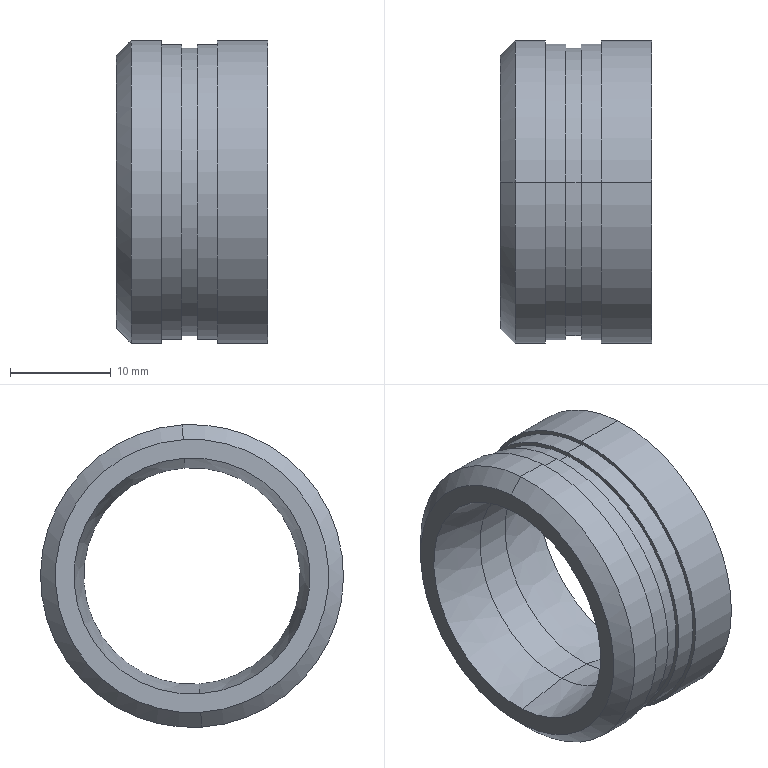Component | SolidWorks | 216InnerTubeAssembly-1_DampingSleeve-1 | 1 solid | 26 faces | box 15 x 30 x 30 mm | volume 4390 mm3 | cylinder 12 | cone 10 | plane 4 | commonest cylinder face diameters 30 x4 29.265 x2 28.514 x2 29.257 x2 21.449 x2 | material Polyurethane(11671)
build123d program:
from build123d import *


with BuildPart() as part:
    # Model → Revolve1 (revolve)
    with BuildSketch(Plane.XY, mode=Mode.PRIVATE) as revolve1_sk:
        Polygon((1.544, 15.169), (0.07655, 13.701), (0.07655, 11.863), (5.577, 10.893), (9.077, 10.893), (15.077, 12.169), (15.077, 15.169), (10.077, 15.169), (10.077, 14.797), (8.077, 14.797), (8.077, 14.426), (6.577, 14.426), (6.578, 14.801), (4.544, 14.801), (4.544, 15.169), align=None)
    revolve(revolve1_sk.sketch.rotate(Axis((0.08037, 0.1686, 0), (1, 0, 0)), 90), axis=Axis((0.08037, 0.1686, 0), (1, 0, 0)))


solid = part.part

# Placed as in the assembly
solid = solid.moved(Location((658.502, -0.1686, 0), (0, 0, 0)))
STEP:
#1=COLOUR_RGB('',0.7922,0.8196,0.9333);
#2=FILL_AREA_STYLE_COLOUR('',#1);
#3=FILL_AREA_STYLE('',(#2));
#4=SURFACE_STYLE_FILL_AREA(#3);
#5=SURFACE_SIDE_STYLE('',(#4));
#6=SURFACE_STYLE_USAGE(.BOTH.,#5);
#7=PRESENTATION_STYLE_ASSIGNMENT((#6));
#8=CARTESIAN_POINT('',(26.104,0.03778,0.5893));
#9=VERTEX_POINT('',#8);
#10=CARTESIAN_POINT('',(26.104,-0.03778,-0.5893));
#11=VERTEX_POINT('',#10);
#12=CARTESIAN_POINT('',(26.104,-0.,0.));
#13=DIRECTION('',(-1.,-0.,0.));
#14=DIRECTION('',(0.,0.06397,0.998));
#15=AXIS2_PLACEMENT_3D('',#12,#13,#14);
#16=CIRCLE('',#15,0.5906);
#17=EDGE_CURVE('',#9,#11,#16,.T.);
#18=ORIENTED_EDGE('',*,*,#17,.T.);
#19=CARTESIAN_POINT('',(25.986,-0.03778,-0.5893));
#20=VERTEX_POINT('',#19);
#21=CARTESIAN_POINT('',(25.928,-0.03778,-0.5893));
#22=DIRECTION('',(-1.,-0.,0.));
#23=VECTOR('',#22,39.37);
#24=LINE('',#21,#23);
#25=EDGE_CURVE('',#11,#20,#24,.T.);
#26=ORIENTED_EDGE('',*,*,#25,.T.);
#27=CARTESIAN_POINT('',(25.986,0.03778,0.5893));
#28=VERTEX_POINT('',#27);
#29=CARTESIAN_POINT('',(25.986,-0.,0.));
#30=DIRECTION('',(-1.,-0.,0.));
#31=DIRECTION('',(0.,0.06397,0.998));
#32=AXIS2_PLACEMENT_3D('',#29,#30,#31);
#33=CIRCLE('',#32,0.5906);
#34=EDGE_CURVE('',#28,#20,#33,.T.);
#35=ORIENTED_EDGE('',*,*,#34,.F.);
#36=CARTESIAN_POINT('',(25.928,0.03778,0.5893));
#37=DIRECTION('',(-1.,-0.,0.));
#38=VECTOR('',#37,39.37);
#39=LINE('',#36,#38);
#40=EDGE_CURVE('',#9,#28,#39,.T.);
#41=ORIENTED_EDGE('',*,*,#40,.F.);
#42=EDGE_LOOP('',(#18,#26,#35,#41));
#43=FACE_OUTER_BOUND('',#42,.T.);
#44=CARTESIAN_POINT('',(25.928,-0.,0.));
#45=DIRECTION('',(-1.,-0.,0.));
#46=DIRECTION('',(0.,0.06397,0.998));
#47=AXIS2_PLACEMENT_3D('',#44,#45,#46);
#48=CYLINDRICAL_SURFACE('',#47,0.5906);
#49=ADVANCED_FACE('',(#43),#48,.T.);
#50=CARTESIAN_POINT('',(26.184,0.03685,0.5749));
#51=VERTEX_POINT('',#50);
#52=CARTESIAN_POINT('',(26.184,-0.03685,-0.5749));
#53=VERTEX_POINT('',#52);
#54=CARTESIAN_POINT('',(26.184,-0.,0.));
#55=DIRECTION('',(-1.,-0.,0.));
#56=DIRECTION('',(0.,0.06397,0.998));
#57=AXIS2_PLACEMENT_3D('',#54,#55,#56);
#58=CIRCLE('',#57,0.5761);
#59=EDGE_CURVE('',#51,#53,#58,.T.);
#60=ORIENTED_EDGE('',*,*,#59,.T.);
#61=CARTESIAN_POINT('',(26.104,-0.03685,-0.5749));
#62=VERTEX_POINT('',#61);
#63=CARTESIAN_POINT('',(25.928,-0.03685,-0.5749));
#64=DIRECTION('',(-1.,-0.,0.));
#65=VECTOR('',#64,39.37);
#66=LINE('',#63,#65);
#67=EDGE_CURVE('',#53,#62,#66,.T.);
#68=ORIENTED_EDGE('',*,*,#67,.T.);
#69=CARTESIAN_POINT('',(26.104,0.03685,0.5749));
#70=VERTEX_POINT('',#69);
#71=CARTESIAN_POINT('',(26.104,-0.,0.));
#72=DIRECTION('',(-1.,-0.,0.));
#73=DIRECTION('',(0.,0.06397,0.998));
#74=AXIS2_PLACEMENT_3D('',#71,#72,#73);
#75=CIRCLE('',#74,0.5761);
#76=EDGE_CURVE('',#70,#62,#75,.T.);
#77=ORIENTED_EDGE('',*,*,#76,.F.);
#78=CARTESIAN_POINT('',(25.928,0.03685,0.5749));
#79=DIRECTION('',(-1.,-0.,0.));
#80=VECTOR('',#79,39.37);
#81=LINE('',#78,#80);
#82=EDGE_CURVE('',#51,#70,#81,.T.);
#83=ORIENTED_EDGE('',*,*,#82,.F.);
#84=EDGE_LOOP('',(#60,#68,#77,#83));
#85=FACE_OUTER_BOUND('',#84,.T.);
#86=CARTESIAN_POINT('',(25.928,-0.,0.));
#87=DIRECTION('',(-1.,-0.,0.));
#88=DIRECTION('',(0.,0.06397,0.998));
#89=AXIS2_PLACEMENT_3D('',#86,#87,#88);
#90=CYLINDRICAL_SURFACE('',#89,0.5761);
#91=ADVANCED_FACE('',(#85),#90,.T.);
#92=CARTESIAN_POINT('',(26.184,-0.03591,-0.5602));
#93=VERTEX_POINT('',#92);
#94=CARTESIAN_POINT('',(26.184,0.03591,0.5602));
#95=VERTEX_POINT('',#94);
#96=CARTESIAN_POINT('',(26.184,-0.,0.));
#97=DIRECTION('',(-1.,-0.,0.));
#98=DIRECTION('',(0.,0.06397,0.998));
#99=AXIS2_PLACEMENT_3D('',#96,#97,#98);
#100=CIRCLE('',#99,0.5613);
#101=EDGE_CURVE('',#93,#95,#100,.T.);
#102=ORIENTED_EDGE('',*,*,#101,.T.);
#103=CARTESIAN_POINT('',(26.184,0.03591,0.5602));
#104=DIRECTION('',(0.001262,0.06397,0.998));
#105=VECTOR('',#104,39.37);
#106=LINE('',#103,#105);
#107=EDGE_CURVE('',#95,#51,#106,.T.);
#108=ORIENTED_EDGE('',*,*,#107,.T.);
#109=CARTESIAN_POINT('',(26.184,-0.,0.));
#110=DIRECTION('',(-1.,-0.,0.));
#111=DIRECTION('',(0.,0.06397,0.998));
#112=AXIS2_PLACEMENT_3D('',#109,#110,#111);
#113=CIRCLE('',#112,0.5761);
#114=EDGE_CURVE('',#53,#51,#113,.T.);
#115=ORIENTED_EDGE('',*,*,#114,.F.);
#116=CARTESIAN_POINT('',(26.184,-0.03591,-0.5602));
#117=DIRECTION('',(0.001262,-0.06397,-0.998));
#118=VECTOR('',#117,39.37);
#119=LINE('',#116,#118);
#120=EDGE_CURVE('',#93,#53,#119,.T.);
#121=ORIENTED_EDGE('',*,*,#120,.F.);
#122=EDGE_LOOP('',(#102,#108,#115,#121));
#123=FACE_OUTER_BOUND('',#122,.T.);
#124=CARTESIAN_POINT('',(26.184,-0.,0.));
#125=DIRECTION('',(1.,0.,-0.));
#126=DIRECTION('',(0.,-0.06397,-0.998));
#127=AXIS2_PLACEMENT_3D('',#124,#125,#126);
#128=CONICAL_SURFACE('',#127,0.5613,1.57);
#129=ADVANCED_FACE('',(#123),#128,.F.);
#130=CARTESIAN_POINT('',(26.243,0.03591,0.5602));
#131=VERTEX_POINT('',#130);
#132=CARTESIAN_POINT('',(26.243,-0.03591,-0.5602));
#133=VERTEX_POINT('',#132);
#134=CARTESIAN_POINT('',(26.243,-0.,0.));
#135=DIRECTION('',(-1.,-0.,0.));
#136=DIRECTION('',(0.,0.06397,0.998));
#137=AXIS2_PLACEMENT_3D('',#134,#135,#136);
#138=CIRCLE('',#137,0.5613);
#139=EDGE_CURVE('',#131,#133,#138,.T.);
#140=ORIENTED_EDGE('',*,*,#139,.T.);
#141=CARTESIAN_POINT('',(25.928,-0.03591,-0.5602));
#142=DIRECTION('',(-1.,-0.,0.));
#143=VECTOR('',#142,39.37);
#144=LINE('',#141,#143);
#145=EDGE_CURVE('',#133,#93,#144,.T.);
#146=ORIENTED_EDGE('',*,*,#145,.T.);
#147=CARTESIAN_POINT('',(26.184,-0.,0.));
#148=DIRECTION('',(-1.,-0.,0.));
#149=DIRECTION('',(0.,0.06397,0.998));
#150=AXIS2_PLACEMENT_3D('',#147,#148,#149);
#151=CIRCLE('',#150,0.5613);
#152=EDGE_CURVE('',#95,#93,#151,.T.);
#153=ORIENTED_EDGE('',*,*,#152,.F.);
#154=CARTESIAN_POINT('',(25.928,0.03591,0.5602));
#155=DIRECTION('',(-1.,-0.,0.));
#156=VECTOR('',#155,39.37);
#157=LINE('',#154,#156);
#158=EDGE_CURVE('',#131,#95,#157,.T.);
#159=ORIENTED_EDGE('',*,*,#158,.F.);
#160=EDGE_LOOP('',(#140,#146,#153,#159));
#161=FACE_OUTER_BOUND('',#160,.T.);
#162=CARTESIAN_POINT('',(25.928,-0.,0.));
#163=DIRECTION('',(-1.,-0.,0.));
#164=DIRECTION('',(0.,0.06397,0.998));
#165=AXIS2_PLACEMENT_3D('',#162,#163,#164);
#166=CYLINDRICAL_SURFACE('',#165,0.5613);
#167=ADVANCED_FACE('',(#161),#166,.T.);
#168=CARTESIAN_POINT('',(26.322,0.03684,0.5747));
#169=VERTEX_POINT('',#168);
#170=CARTESIAN_POINT('',(26.322,-0.03684,-0.5747));
#171=VERTEX_POINT('',#170);
#172=CARTESIAN_POINT('',(26.322,-0.,0.));
#173=DIRECTION('',(-1.,-0.,0.));
#174=DIRECTION('',(0.,0.06397,0.998));
#175=AXIS2_PLACEMENT_3D('',#172,#173,#174);
#176=CIRCLE('',#175,0.5759);
#177=EDGE_CURVE('',#169,#171,#176,.T.);
#178=ORIENTED_EDGE('',*,*,#177,.T.);
#179=CARTESIAN_POINT('',(26.243,-0.03684,-0.5747));
#180=VERTEX_POINT('',#179);
#181=CARTESIAN_POINT('',(25.928,-0.03684,-0.5747));
#182=DIRECTION('',(-1.,-0.,0.));
#183=VECTOR('',#182,39.37);
#184=LINE('',#181,#183);
#185=EDGE_CURVE('',#171,#180,#184,.T.);
#186=ORIENTED_EDGE('',*,*,#185,.T.);
#187=CARTESIAN_POINT('',(26.243,0.03684,0.5747));
#188=VERTEX_POINT('',#187);
#189=CARTESIAN_POINT('',(26.243,-0.,0.));
#190=DIRECTION('',(-1.,-0.,0.));
#191=DIRECTION('',(0.,0.06397,0.998));
#192=AXIS2_PLACEMENT_3D('',#189,#190,#191);
#193=CIRCLE('',#192,0.5759);
#194=EDGE_CURVE('',#188,#180,#193,.T.);
#195=ORIENTED_EDGE('',*,*,#194,.F.);
#196=CARTESIAN_POINT('',(25.928,0.03684,0.5747));
#197=DIRECTION('',(-1.,-0.,0.));
#198=VECTOR('',#197,39.37);
#199=LINE('',#196,#198);
#200=EDGE_CURVE('',#169,#188,#199,.T.);
#201=ORIENTED_EDGE('',*,*,#200,.F.);
#202=EDGE_LOOP('',(#178,#186,#195,#201));
#203=FACE_OUTER_BOUND('',#202,.T.);
#204=CARTESIAN_POINT('',(25.928,-0.,0.));
#205=DIRECTION('',(-1.,-0.,0.));
#206=DIRECTION('',(0.,0.06397,0.998));
#207=AXIS2_PLACEMENT_3D('',#204,#205,#206);
#208=CYLINDRICAL_SURFACE('',#207,0.5759);
#209=ADVANCED_FACE('',(#203),#208,.T.);
#210=CARTESIAN_POINT('',(26.322,-0.,0.));
#211=DIRECTION('',(-1.,-0.,0.));
#212=DIRECTION('',(0.,0.06397,0.998));
#213=AXIS2_PLACEMENT_3D('',#210,#211,#212);
#214=CIRCLE('',#213,0.5759);
#215=EDGE_CURVE('',#171,#169,#214,.T.);
#216=ORIENTED_EDGE('',*,*,#215,.F.);
#217=CARTESIAN_POINT('',(26.322,-0.03778,-0.5893));
#218=VERTEX_POINT('',#217);
#219=CARTESIAN_POINT('',(26.322,-0.03684,-0.5747));
#220=DIRECTION('',(-0.002523,-0.06397,-0.9979));
#221=VECTOR('',#220,39.37);
#222=LINE('',#219,#221);
#223=EDGE_CURVE('',#171,#218,#222,.T.);
#224=ORIENTED_EDGE('',*,*,#223,.T.);
#225=CARTESIAN_POINT('',(26.322,0.03778,0.5893));
#226=VERTEX_POINT('',#225);
#227=CARTESIAN_POINT('',(26.322,-0.,0.));
#228=DIRECTION('',(-1.,-0.,0.));
#229=DIRECTION('',(0.,0.06397,0.998));
#230=AXIS2_PLACEMENT_3D('',#227,#228,#229);
#231=CIRCLE('',#230,0.5906);
#232=EDGE_CURVE('',#218,#226,#231,.T.);
#233=ORIENTED_EDGE('',*,*,#232,.T.);
#234=CARTESIAN_POINT('',(26.322,0.03684,0.5747));
#235=DIRECTION('',(-0.002523,0.06397,0.9979));
#236=VECTOR('',#235,39.37);
#237=LINE('',#234,#236);
#238=EDGE_CURVE('',#169,#226,#237,.T.);
#239=ORIENTED_EDGE('',*,*,#238,.F.);
#240=EDGE_LOOP('',(#216,#224,#233,#239));
#241=FACE_OUTER_BOUND('',#240,.T.);
#242=CARTESIAN_POINT('',(26.322,-0.,0.));
#243=DIRECTION('',(-1.,-0.,0.));
#244=DIRECTION('',(0.,0.06397,0.998));
#245=AXIS2_PLACEMENT_3D('',#242,#243,#244);
#246=CONICAL_SURFACE('',#245,0.5759,1.568);
#247=ADVANCED_FACE('',(#241),#246,.F.);
#248=CARTESIAN_POINT('',(26.519,0.03778,0.5893));
#249=VERTEX_POINT('',#248);
#250=CARTESIAN_POINT('',(26.519,-0.03778,-0.5893));
#251=VERTEX_POINT('',#250);
#252=CARTESIAN_POINT('',(26.519,-0.,0.));
#253=DIRECTION('',(-1.,-0.,0.));
#254=DIRECTION('',(0.,0.06397,0.998));
#255=AXIS2_PLACEMENT_3D('',#252,#253,#254);
#256=CIRCLE('',#255,0.5906);
#257=EDGE_CURVE('',#249,#251,#256,.T.);
#258=ORIENTED_EDGE('',*,*,#257,.T.);
#259=CARTESIAN_POINT('',(25.928,-0.03778,-0.5893));
#260=DIRECTION('',(-1.,-0.,0.));
#261=VECTOR('',#260,39.37);
#262=LINE('',#259,#261);
#263=EDGE_CURVE('',#251,#218,#262,.T.);
#264=ORIENTED_EDGE('',*,*,#263,.T.);
#265=CARTESIAN_POINT('',(26.322,-0.,0.));
#266=DIRECTION('',(-1.,-0.,0.));
#267=DIRECTION('',(0.,0.06397,0.998));
#268=AXIS2_PLACEMENT_3D('',#265,#266,#267);
#269=CIRCLE('',#268,0.5906);
#270=EDGE_CURVE('',#226,#218,#269,.T.);
#271=ORIENTED_EDGE('',*,*,#270,.F.);
#272=CARTESIAN_POINT('',(25.928,0.03778,0.5893));
#273=DIRECTION('',(-1.,-0.,0.));
#274=VECTOR('',#273,39.37);
#275=LINE('',#272,#274);
#276=EDGE_CURVE('',#249,#226,#275,.T.);
#277=ORIENTED_EDGE('',*,*,#276,.F.);
#278=EDGE_LOOP('',(#258,#264,#271,#277));
#279=FACE_OUTER_BOUND('',#278,.T.);
#280=CARTESIAN_POINT('',(25.928,-0.,0.));
#281=DIRECTION('',(-1.,-0.,0.));
#282=DIRECTION('',(0.,0.06397,0.998));
#283=AXIS2_PLACEMENT_3D('',#280,#281,#282);
#284=CYLINDRICAL_SURFACE('',#283,0.5906);
#285=ADVANCED_FACE('',(#279),#284,.T.);
#286=CARTESIAN_POINT('',(26.283,-0.02701,-0.4214));
#287=VERTEX_POINT('',#286);
#288=CARTESIAN_POINT('',(26.283,0.02701,0.4214));
#289=VERTEX_POINT('',#288);
#290=CARTESIAN_POINT('',(26.283,-0.,0.));
#291=DIRECTION('',(-1.,-0.,0.));
#292=DIRECTION('',(0.,0.06397,0.998));
#293=AXIS2_PLACEMENT_3D('',#290,#291,#292);
#294=CIRCLE('',#293,0.4222);
#295=EDGE_CURVE('',#287,#289,#294,.T.);
#296=ORIENTED_EDGE('',*,*,#295,.T.);
#297=CARTESIAN_POINT('',(26.519,0.03022,0.4715));
#298=VERTEX_POINT('',#297);
#299=CARTESIAN_POINT('',(26.519,0.03022,0.4715));
#300=DIRECTION('',(0.9781,0.0133,0.2075));
#301=VECTOR('',#300,39.37);
#302=LINE('',#299,#301);
#303=EDGE_CURVE('',#289,#298,#302,.T.);
#304=ORIENTED_EDGE('',*,*,#303,.T.);
#305=CARTESIAN_POINT('',(26.519,-0.03022,-0.4715));
#306=VERTEX_POINT('',#305);
#307=CARTESIAN_POINT('',(26.519,-0.,0.));
#308=DIRECTION('',(-1.,-0.,0.));
#309=DIRECTION('',(0.,0.06397,0.998));
#310=AXIS2_PLACEMENT_3D('',#307,#308,#309);
#311=CIRCLE('',#310,0.4724);
#312=EDGE_CURVE('',#306,#298,#311,.T.);
#313=ORIENTED_EDGE('',*,*,#312,.F.);
#314=CARTESIAN_POINT('',(26.519,-0.03022,-0.4715));
#315=DIRECTION('',(0.9781,-0.0133,-0.2075));
#316=VECTOR('',#315,39.37);
#317=LINE('',#314,#316);
#318=EDGE_CURVE('',#287,#306,#317,.T.);
#319=ORIENTED_EDGE('',*,*,#318,.F.);
#320=EDGE_LOOP('',(#296,#304,#313,#319));
#321=FACE_OUTER_BOUND('',#320,.T.);
#322=CARTESIAN_POINT('',(26.519,-0.,0.));
#323=DIRECTION('',(1.,0.,-0.));
#324=DIRECTION('',(0.,-0.06397,-0.998));
#325=AXIS2_PLACEMENT_3D('',#322,#323,#324);
#326=CONICAL_SURFACE('',#325,0.4724,0.2094);
#327=ADVANCED_FACE('',(#321),#326,.F.);
#328=ORIENTED_EDGE('',*,*,#295,.F.);
#329=CARTESIAN_POINT('',(26.145,-0.02701,-0.4214));
#330=VERTEX_POINT('',#329);
#331=CARTESIAN_POINT('',(25.928,-0.02701,-0.4214));
#332=DIRECTION('',(-1.,-0.,0.));
#333=VECTOR('',#332,39.37);
#334=LINE('',#331,#333);
#335=EDGE_CURVE('',#287,#330,#334,.T.);
#336=ORIENTED_EDGE('',*,*,#335,.T.);
#337=CARTESIAN_POINT('',(26.145,0.02701,0.4214));
#338=VERTEX_POINT('',#337);
#339=CARTESIAN_POINT('',(26.145,-0.,0.));
#340=DIRECTION('',(-1.,-0.,0.));
#341=DIRECTION('',(0.,0.06397,0.998));
#342=AXIS2_PLACEMENT_3D('',#339,#340,#341);
#343=CIRCLE('',#342,0.4222);
#344=EDGE_CURVE('',#330,#338,#343,.T.);
#345=ORIENTED_EDGE('',*,*,#344,.T.);
#346=CARTESIAN_POINT('',(25.928,0.02701,0.4214));
#347=DIRECTION('',(-1.,-0.,0.));
#348=VECTOR('',#347,39.37);
#349=LINE('',#346,#348);
#350=EDGE_CURVE('',#289,#338,#349,.T.);
#351=ORIENTED_EDGE('',*,*,#350,.F.);
#352=EDGE_LOOP('',(#328,#336,#345,#351));
#353=FACE_OUTER_BOUND('',#352,.T.);
#354=CARTESIAN_POINT('',(25.928,-0.,0.));
#355=DIRECTION('',(-1.,-0.,0.));
#356=DIRECTION('',(0.,0.06397,0.998));
#357=AXIS2_PLACEMENT_3D('',#354,#355,#356);
#358=CYLINDRICAL_SURFACE('',#357,0.4222);
#359=ADVANCED_FACE('',(#353),#358,.F.);
#360=ORIENTED_EDGE('',*,*,#344,.F.);
#361=CARTESIAN_POINT('',(25.928,-0.02945,-0.4595));
#362=VERTEX_POINT('',#361);
#363=CARTESIAN_POINT('',(25.928,-0.02945,-0.4595));
#364=DIRECTION('',(-0.9848,-0.01111,-0.1733));
#365=VECTOR('',#364,39.37);
#366=LINE('',#363,#365);
#367=EDGE_CURVE('',#330,#362,#366,.T.);
#368=ORIENTED_EDGE('',*,*,#367,.T.);
#369=CARTESIAN_POINT('',(25.928,0.02945,0.4595));
#370=VERTEX_POINT('',#369);
#371=CARTESIAN_POINT('',(25.928,-0.,0.));
#372=DIRECTION('',(-1.,-0.,0.));
#373=DIRECTION('',(0.,0.06397,0.998));
#374=AXIS2_PLACEMENT_3D('',#371,#372,#373);
#375=CIRCLE('',#374,0.4604);
#376=EDGE_CURVE('',#362,#370,#375,.T.);
#377=ORIENTED_EDGE('',*,*,#376,.T.);
#378=CARTESIAN_POINT('',(25.928,0.02945,0.4595));
#379=DIRECTION('',(-0.9848,0.01111,0.1733));
#380=VECTOR('',#379,39.37);
#381=LINE('',#378,#380);
#382=EDGE_CURVE('',#338,#370,#381,.T.);
#383=ORIENTED_EDGE('',*,*,#382,.F.);
#384=EDGE_LOOP('',(#360,#368,#377,#383));
#385=FACE_OUTER_BOUND('',#384,.T.);
#386=CARTESIAN_POINT('',(25.928,-0.,0.));
#387=DIRECTION('',(-1.,-0.,0.));
#388=DIRECTION('',(0.,0.06397,0.998));
#389=AXIS2_PLACEMENT_3D('',#386,#387,#388);
#390=CONICAL_SURFACE('',#389,0.4604,0.1745);
#391=ADVANCED_FACE('',(#385),#390,.F.);
#392=CARTESIAN_POINT('',(25.928,0.03408,0.5317));
#393=VERTEX_POINT('',#392);
#394=CARTESIAN_POINT('',(25.928,-0.03408,-0.5317));
#395=VERTEX_POINT('',#394);
#396=CARTESIAN_POINT('',(25.928,-0.,0.));
#397=DIRECTION('',(-1.,-0.,0.));
#398=DIRECTION('',(0.,0.06397,0.998));
#399=AXIS2_PLACEMENT_3D('',#396,#397,#398);
#400=CIRCLE('',#399,0.5328);
#401=EDGE_CURVE('',#393,#395,#400,.T.);
#402=ORIENTED_EDGE('',*,*,#401,.F.);
#403=CARTESIAN_POINT('',(25.986,0.03778,0.5893));
#404=DIRECTION('',(0.7071,0.04523,0.7056));
#405=VECTOR('',#404,39.37);
#406=LINE('',#403,#405);
#407=EDGE_CURVE('',#393,#28,#406,.T.);
#408=ORIENTED_EDGE('',*,*,#407,.T.);
#409=ORIENTED_EDGE('',*,*,#34,.T.);
#410=CARTESIAN_POINT('',(25.986,-0.03778,-0.5893));
#411=DIRECTION('',(0.7071,-0.04523,-0.7056));
#412=VECTOR('',#411,39.37);
#413=LINE('',#410,#412);
#414=EDGE_CURVE('',#395,#20,#413,.T.);
#415=ORIENTED_EDGE('',*,*,#414,.F.);
#416=EDGE_LOOP('',(#402,#408,#409,#415));
#417=FACE_OUTER_BOUND('',#416,.T.);
#418=CARTESIAN_POINT('',(25.986,-0.,0.));
#419=DIRECTION('',(1.,0.,-0.));
#420=DIRECTION('',(0.,-0.06397,-0.998));
#421=AXIS2_PLACEMENT_3D('',#418,#419,#420);
#422=CONICAL_SURFACE('',#421,0.5906,0.7854);
#423=ADVANCED_FACE('',(#417),#422,.T.);
#424=ORIENTED_EDGE('',*,*,#407,.F.);
#425=CARTESIAN_POINT('',(25.928,-0.,0.));
#426=DIRECTION('',(-1.,-0.,0.));
#427=DIRECTION('',(0.,0.06397,0.998));
#428=AXIS2_PLACEMENT_3D('',#425,#426,#427);
#429=CIRCLE('',#428,0.5328);
#430=EDGE_CURVE('',#395,#393,#429,.T.);
#431=ORIENTED_EDGE('',*,*,#430,.F.);
#432=ORIENTED_EDGE('',*,*,#414,.T.);
#433=CARTESIAN_POINT('',(25.986,-0.,0.));
#434=DIRECTION('',(-1.,-0.,0.));
#435=DIRECTION('',(0.,0.06397,0.998));
#436=AXIS2_PLACEMENT_3D('',#433,#434,#435);
#437=CIRCLE('',#436,0.5906);
#438=EDGE_CURVE('',#20,#28,#437,.T.);
#439=ORIENTED_EDGE('',*,*,#438,.T.);
#440=EDGE_LOOP('',(#424,#431,#432,#439));
#441=FACE_OUTER_BOUND('',#440,.T.);
#442=CARTESIAN_POINT('',(25.986,-0.,0.));
#443=DIRECTION('',(1.,0.,-0.));
#444=DIRECTION('',(0.,-0.06397,-0.998));
#445=AXIS2_PLACEMENT_3D('',#442,#443,#444);
#446=CONICAL_SURFACE('',#445,0.5906,0.7854);
#447=ADVANCED_FACE('',(#441),#446,.T.);
#448=CARTESIAN_POINT('',(25.928,-0.,0.));
#449=DIRECTION('',(-1.,-0.,0.));
#450=DIRECTION('',(0.,0.06397,0.998));
#451=AXIS2_PLACEMENT_3D('',#448,#449,#450);
#452=CIRCLE('',#451,0.4604);
#453=EDGE_CURVE('',#370,#362,#452,.T.);
#454=ORIENTED_EDGE('',*,*,#453,.F.);
#455=ORIENTED_EDGE('',*,*,#376,.F.);
#456=EDGE_LOOP('',(#454,#455));
#457=FACE_BOUND('',#456,.T.);
#458=ORIENTED_EDGE('',*,*,#430,.T.);
#459=ORIENTED_EDGE('',*,*,#401,.T.);
#460=EDGE_LOOP('',(#458,#459));
#461=FACE_OUTER_BOUND('',#460,.T.);
#462=CARTESIAN_POINT('',(25.928,-0.006626,0.0004247));
#463=DIRECTION('',(1.,0.,-0.));
#464=DIRECTION('',(-0.,-0.06397,-0.998));
#465=AXIS2_PLACEMENT_3D('',#462,#463,#464);
#466=PLANE('',#465);
#467=ADVANCED_FACE('',(#457,#461),#466,.F.);
#468=ORIENTED_EDGE('',*,*,#367,.F.);
#469=CARTESIAN_POINT('',(26.145,-0.,0.));
#470=DIRECTION('',(-1.,-0.,0.));
#471=DIRECTION('',(0.,0.06397,0.998));
#472=AXIS2_PLACEMENT_3D('',#469,#470,#471);
#473=CIRCLE('',#472,0.4222);
#474=EDGE_CURVE('',#338,#330,#473,.T.);
#475=ORIENTED_EDGE('',*,*,#474,.F.);
#476=ORIENTED_EDGE('',*,*,#382,.T.);
#477=ORIENTED_EDGE('',*,*,#453,.T.);
#478=EDGE_LOOP('',(#468,#475,#476,#477));
#479=FACE_OUTER_BOUND('',#478,.T.);
#480=CARTESIAN_POINT('',(25.928,-0.,0.));
#481=DIRECTION('',(-1.,-0.,0.));
#482=DIRECTION('',(0.,0.06397,0.998));
#483=AXIS2_PLACEMENT_3D('',#480,#481,#482);
#484=CONICAL_SURFACE('',#483,0.4604,0.1745);
#485=ADVANCED_FACE('',(#479),#484,.F.);
#486=ORIENTED_EDGE('',*,*,#335,.F.);
#487=CARTESIAN_POINT('',(26.283,-0.,0.));
#488=DIRECTION('',(-1.,-0.,0.));
#489=DIRECTION('',(0.,0.06397,0.998));
#490=AXIS2_PLACEMENT_3D('',#487,#488,#489);
#491=CIRCLE('',#490,0.4222);
#492=EDGE_CURVE('',#289,#287,#491,.T.);
#493=ORIENTED_EDGE('',*,*,#492,.F.);
#494=ORIENTED_EDGE('',*,*,#350,.T.);
#495=ORIENTED_EDGE('',*,*,#474,.T.);
#496=EDGE_LOOP('',(#486,#493,#494,#495));
#497=FACE_OUTER_BOUND('',#496,.T.);
#498=CARTESIAN_POINT('',(25.928,-0.,0.));
#499=DIRECTION('',(-1.,-0.,0.));
#500=DIRECTION('',(0.,0.06397,0.998));
#501=AXIS2_PLACEMENT_3D('',#498,#499,#500);
#502=CYLINDRICAL_SURFACE('',#501,0.4222);
#503=ADVANCED_FACE('',(#497),#502,.F.);
#504=ORIENTED_EDGE('',*,*,#303,.F.);
#505=ORIENTED_EDGE('',*,*,#492,.T.);
#506=ORIENTED_EDGE('',*,*,#318,.T.);
#507=CARTESIAN_POINT('',(26.519,-0.,0.));
#508=DIRECTION('',(-1.,-0.,0.));
#509=DIRECTION('',(0.,0.06397,0.998));
#510=AXIS2_PLACEMENT_3D('',#507,#508,#509);
#511=CIRCLE('',#510,0.4724);
#512=EDGE_CURVE('',#298,#306,#511,.T.);
#513=ORIENTED_EDGE('',*,*,#512,.F.);
#514=EDGE_LOOP('',(#504,#505,#506,#513));
#515=FACE_OUTER_BOUND('',#514,.T.);
#516=CARTESIAN_POINT('',(26.519,-0.,0.));
#517=DIRECTION('',(1.,0.,-0.));
#518=DIRECTION('',(0.,-0.06397,-0.998));
#519=AXIS2_PLACEMENT_3D('',#516,#517,#518);
#520=CONICAL_SURFACE('',#519,0.4724,0.2094);
#521=ADVANCED_FACE('',(#515),#520,.F.);
#522=ORIENTED_EDGE('',*,*,#257,.F.);
#523=CARTESIAN_POINT('',(26.519,-0.,0.));
#524=DIRECTION('',(-1.,-0.,0.));
#525=DIRECTION('',(0.,0.06397,0.998));
#526=AXIS2_PLACEMENT_3D('',#523,#524,#525);
#527=CIRCLE('',#526,0.5906);
#528=EDGE_CURVE('',#251,#249,#527,.T.);
#529=ORIENTED_EDGE('',*,*,#528,.F.);
#530=EDGE_LOOP('',(#522,#529));
#531=FACE_OUTER_BOUND('',#530,.T.);
#532=ORIENTED_EDGE('',*,*,#312,.T.);
#533=ORIENTED_EDGE('',*,*,#512,.T.);
#534=EDGE_LOOP('',(#532,#533));
#535=FACE_BOUND('',#534,.T.);
#536=CARTESIAN_POINT('',(26.519,-0.006626,0.0004247));
#537=DIRECTION('',(-1.,-0.,0.));
#538=DIRECTION('',(0.,0.06397,0.998));
#539=AXIS2_PLACEMENT_3D('',#536,#537,#538);
#540=PLANE('',#539);
#541=ADVANCED_FACE('',(#531,#535),#540,.F.);
#542=ORIENTED_EDGE('',*,*,#263,.F.);
#543=ORIENTED_EDGE('',*,*,#528,.T.);
#544=ORIENTED_EDGE('',*,*,#276,.T.);
#545=ORIENTED_EDGE('',*,*,#232,.F.);
#546=EDGE_LOOP('',(#542,#543,#544,#545));
#547=FACE_OUTER_BOUND('',#546,.T.);
#548=CARTESIAN_POINT('',(25.928,-0.,0.));
#549=DIRECTION('',(-1.,-0.,0.));
#550=DIRECTION('',(0.,0.06397,0.998));
#551=AXIS2_PLACEMENT_3D('',#548,#549,#550);
#552=CYLINDRICAL_SURFACE('',#551,0.5906);
#553=ADVANCED_FACE('',(#547),#552,.T.);
#554=ORIENTED_EDGE('',*,*,#223,.F.);
#555=ORIENTED_EDGE('',*,*,#177,.F.);
#556=ORIENTED_EDGE('',*,*,#238,.T.);
#557=ORIENTED_EDGE('',*,*,#270,.T.);
#558=EDGE_LOOP('',(#554,#555,#556,#557));
#559=FACE_OUTER_BOUND('',#558,.T.);
#560=CARTESIAN_POINT('',(26.322,-0.,0.));
#561=DIRECTION('',(-1.,-0.,0.));
#562=DIRECTION('',(0.,0.06397,0.998));
#563=AXIS2_PLACEMENT_3D('',#560,#561,#562);
#564=CONICAL_SURFACE('',#563,0.5759,1.568);
#565=ADVANCED_FACE('',(#559),#564,.F.);
#566=ORIENTED_EDGE('',*,*,#185,.F.);
#567=ORIENTED_EDGE('',*,*,#215,.T.);
#568=ORIENTED_EDGE('',*,*,#200,.T.);
#569=CARTESIAN_POINT('',(26.243,-0.,0.));
#570=DIRECTION('',(-1.,-0.,0.));
#571=DIRECTION('',(0.,0.06397,0.998));
#572=AXIS2_PLACEMENT_3D('',#569,#570,#571);
#573=CIRCLE('',#572,0.5759);
#574=EDGE_CURVE('',#180,#188,#573,.T.);
#575=ORIENTED_EDGE('',*,*,#574,.F.);
#576=EDGE_LOOP('',(#566,#567,#568,#575));
#577=FACE_OUTER_BOUND('',#576,.T.);
#578=CARTESIAN_POINT('',(25.928,-0.,0.));
#579=DIRECTION('',(-1.,-0.,0.));
#580=DIRECTION('',(0.,0.06397,0.998));
#581=AXIS2_PLACEMENT_3D('',#578,#579,#580);
#582=CYLINDRICAL_SURFACE('',#581,0.5759);
#583=ADVANCED_FACE('',(#577),#582,.T.);
#584=ORIENTED_EDGE('',*,*,#194,.T.);
#585=ORIENTED_EDGE('',*,*,#574,.T.);
#586=EDGE_LOOP('',(#584,#585));
#587=FACE_OUTER_BOUND('',#586,.T.);
#588=ORIENTED_EDGE('',*,*,#139,.F.);
#589=CARTESIAN_POINT('',(26.243,-0.,0.));
#590=DIRECTION('',(-1.,-0.,0.));
#591=DIRECTION('',(0.,0.06397,0.998));
#592=AXIS2_PLACEMENT_3D('',#589,#590,#591);
#593=CIRCLE('',#592,0.5613);
#594=EDGE_CURVE('',#133,#131,#593,.T.);
#595=ORIENTED_EDGE('',*,*,#594,.F.);
#596=EDGE_LOOP('',(#588,#595));
#597=FACE_BOUND('',#596,.T.);
#598=CARTESIAN_POINT('',(26.243,-0.006626,0.0004247));
#599=DIRECTION('',(-1.,-0.,0.));
#600=DIRECTION('',(0.,0.06397,0.998));
#601=AXIS2_PLACEMENT_3D('',#598,#599,#600);
#602=PLANE('',#601);
#603=ADVANCED_FACE('',(#587,#597),#602,.T.);
#604=ORIENTED_EDGE('',*,*,#145,.F.);
#605=ORIENTED_EDGE('',*,*,#594,.T.);
#606=ORIENTED_EDGE('',*,*,#158,.T.);
#607=ORIENTED_EDGE('',*,*,#101,.F.);
#608=EDGE_LOOP('',(#604,#605,#606,#607));
#609=FACE_OUTER_BOUND('',#608,.T.);
#610=CARTESIAN_POINT('',(25.928,-0.,0.));
#611=DIRECTION('',(-1.,-0.,0.));
#612=DIRECTION('',(0.,0.06397,0.998));
#613=AXIS2_PLACEMENT_3D('',#610,#611,#612);
#614=CYLINDRICAL_SURFACE('',#613,0.5613);
#615=ADVANCED_FACE('',(#609),#614,.T.);
#616=ORIENTED_EDGE('',*,*,#107,.F.);
#617=ORIENTED_EDGE('',*,*,#152,.T.);
#618=ORIENTED_EDGE('',*,*,#120,.T.);
#619=ORIENTED_EDGE('',*,*,#59,.F.);
#620=EDGE_LOOP('',(#616,#617,#618,#619));
#621=FACE_OUTER_BOUND('',#620,.T.);
#622=CARTESIAN_POINT('',(26.184,-0.,0.));
#623=DIRECTION('',(1.,0.,-0.));
#624=DIRECTION('',(0.,-0.06397,-0.998));
#625=AXIS2_PLACEMENT_3D('',#622,#623,#624);
#626=CONICAL_SURFACE('',#625,0.5613,1.57);
#627=ADVANCED_FACE('',(#621),#626,.F.);
#628=ORIENTED_EDGE('',*,*,#67,.F.);
#629=ORIENTED_EDGE('',*,*,#114,.T.);
#630=ORIENTED_EDGE('',*,*,#82,.T.);
#631=CARTESIAN_POINT('',(26.104,-0.,0.));
#632=DIRECTION('',(-1.,-0.,0.));
#633=DIRECTION('',(0.,0.06397,0.998));
#634=AXIS2_PLACEMENT_3D('',#631,#632,#633);
#635=CIRCLE('',#634,0.5761);
#636=EDGE_CURVE('',#62,#70,#635,.T.);
#637=ORIENTED_EDGE('',*,*,#636,.F.);
#638=EDGE_LOOP('',(#628,#629,#630,#637));
#639=FACE_OUTER_BOUND('',#638,.T.);
#640=CARTESIAN_POINT('',(25.928,-0.,0.));
#641=DIRECTION('',(-1.,-0.,0.));
#642=DIRECTION('',(0.,0.06397,0.998));
#643=AXIS2_PLACEMENT_3D('',#640,#641,#642);
#644=CYLINDRICAL_SURFACE('',#643,0.5761);
#645=ADVANCED_FACE('',(#639),#644,.T.);
#646=ORIENTED_EDGE('',*,*,#17,.F.);
#647=CARTESIAN_POINT('',(26.104,-0.,0.));
#648=DIRECTION('',(-1.,-0.,0.));
#649=DIRECTION('',(0.,0.06397,0.998));
#650=AXIS2_PLACEMENT_3D('',#647,#648,#649);
#651=CIRCLE('',#650,0.5906);
#652=EDGE_CURVE('',#11,#9,#651,.T.);
#653=ORIENTED_EDGE('',*,*,#652,.F.);
#654=EDGE_LOOP('',(#646,#653));
#655=FACE_OUTER_BOUND('',#654,.T.);
#656=ORIENTED_EDGE('',*,*,#76,.T.);
#657=ORIENTED_EDGE('',*,*,#636,.T.);
#658=EDGE_LOOP('',(#656,#657));
#659=FACE_BOUND('',#658,.T.);
#660=CARTESIAN_POINT('',(26.104,-0.006626,0.0004247));
#661=DIRECTION('',(-1.,-0.,0.));
#662=DIRECTION('',(0.,0.06397,0.998));
#663=AXIS2_PLACEMENT_3D('',#660,#661,#662);
#664=PLANE('',#663);
#665=ADVANCED_FACE('',(#655,#659),#664,.F.);
#666=ORIENTED_EDGE('',*,*,#25,.F.);
#667=ORIENTED_EDGE('',*,*,#652,.T.);
#668=ORIENTED_EDGE('',*,*,#40,.T.);
#669=ORIENTED_EDGE('',*,*,#438,.F.);
#670=EDGE_LOOP('',(#666,#667,#668,#669));
#671=FACE_OUTER_BOUND('',#670,.T.);
#672=CARTESIAN_POINT('',(25.928,-0.,0.));
#673=DIRECTION('',(-1.,-0.,0.));
#674=DIRECTION('',(0.,0.06397,0.998));
#675=AXIS2_PLACEMENT_3D('',#672,#673,#674);
#676=CYLINDRICAL_SURFACE('',#675,0.5906);
#677=ADVANCED_FACE('',(#671),#676,.T.);
#678=CLOSED_SHELL('',(#49,#91,#129,#167,#209,#247,#285,#327,#359,#391,#423,#447,#467,#485,#503,#521,#541,#553,#565,#583,#603,#615,#627,#645,#665,#677));
#679=MANIFOLD_SOLID_BREP('',#678);
#680=STYLED_ITEM('',(#7),#679);
#681=PRESENTATION_LAYER_ASSIGNMENT('','',(#680));
#682=(LENGTH_UNIT()NAMED_UNIT(*)SI_UNIT($,.METRE.));
#683=LENGTH_MEASURE_WITH_UNIT(LENGTH_MEASURE(0.0254),#682);
#684=DIMENSIONAL_EXPONENTS(1.,0.,0.,0.,0.,0.,0.);
#685=(CONVERSION_BASED_UNIT('',#683)LENGTH_UNIT()NAMED_UNIT(#684));
#686=UNCERTAINTY_MEASURE_WITH_UNIT(LENGTH_MEASURE(0.00001),#685,'','');
#687=(NAMED_UNIT(*)PLANE_ANGLE_UNIT()SI_UNIT($,.RADIAN.));
#688=(NAMED_UNIT(*)SI_UNIT($,.STERADIAN.)SOLID_ANGLE_UNIT());
#689=(GEOMETRIC_REPRESENTATION_CONTEXT(3)GLOBAL_UNCERTAINTY_ASSIGNED_CONTEXT((#686))GLOBAL_UNIT_ASSIGNED_CONTEXT((#685,#687,#688))REPRESENTATION_CONTEXT('',''));
#690=MECHANICAL_DESIGN_GEOMETRIC_PRESENTATION_REPRESENTATION('',(#680),#689);
#691=CARTESIAN_POINT('',(0.,0.,0.));
#692=DIRECTION('',(0.,0.,1.));
#693=DIRECTION('',(1.,0.,0.));
#694=AXIS2_PLACEMENT_3D('',#691,#692,#693);
#695=(LENGTH_UNIT()NAMED_UNIT(*)SI_UNIT($,.METRE.));
#696=LENGTH_MEASURE_WITH_UNIT(LENGTH_MEASURE(0.0254),#695);
#697=DIMENSIONAL_EXPONENTS(1.,0.,0.,0.,0.,0.,0.);
#698=(CONVERSION_BASED_UNIT('',#696)LENGTH_UNIT()NAMED_UNIT(#697));
#699=UNCERTAINTY_MEASURE_WITH_UNIT(LENGTH_MEASURE(0.00001),#698,'','');
#700=(NAMED_UNIT(*)PLANE_ANGLE_UNIT()SI_UNIT($,.RADIAN.));
#701=(NAMED_UNIT(*)SI_UNIT($,.STERADIAN.)SOLID_ANGLE_UNIT());
#702=(GEOMETRIC_REPRESENTATION_CONTEXT(3)GLOBAL_UNCERTAINTY_ASSIGNED_CONTEXT((#699))GLOBAL_UNIT_ASSIGNED_CONTEXT((#698,#700,#701))REPRESENTATION_CONTEXT('',''));
#703=ADVANCED_BREP_SHAPE_REPRESENTATION('',(#679,#694),#702);